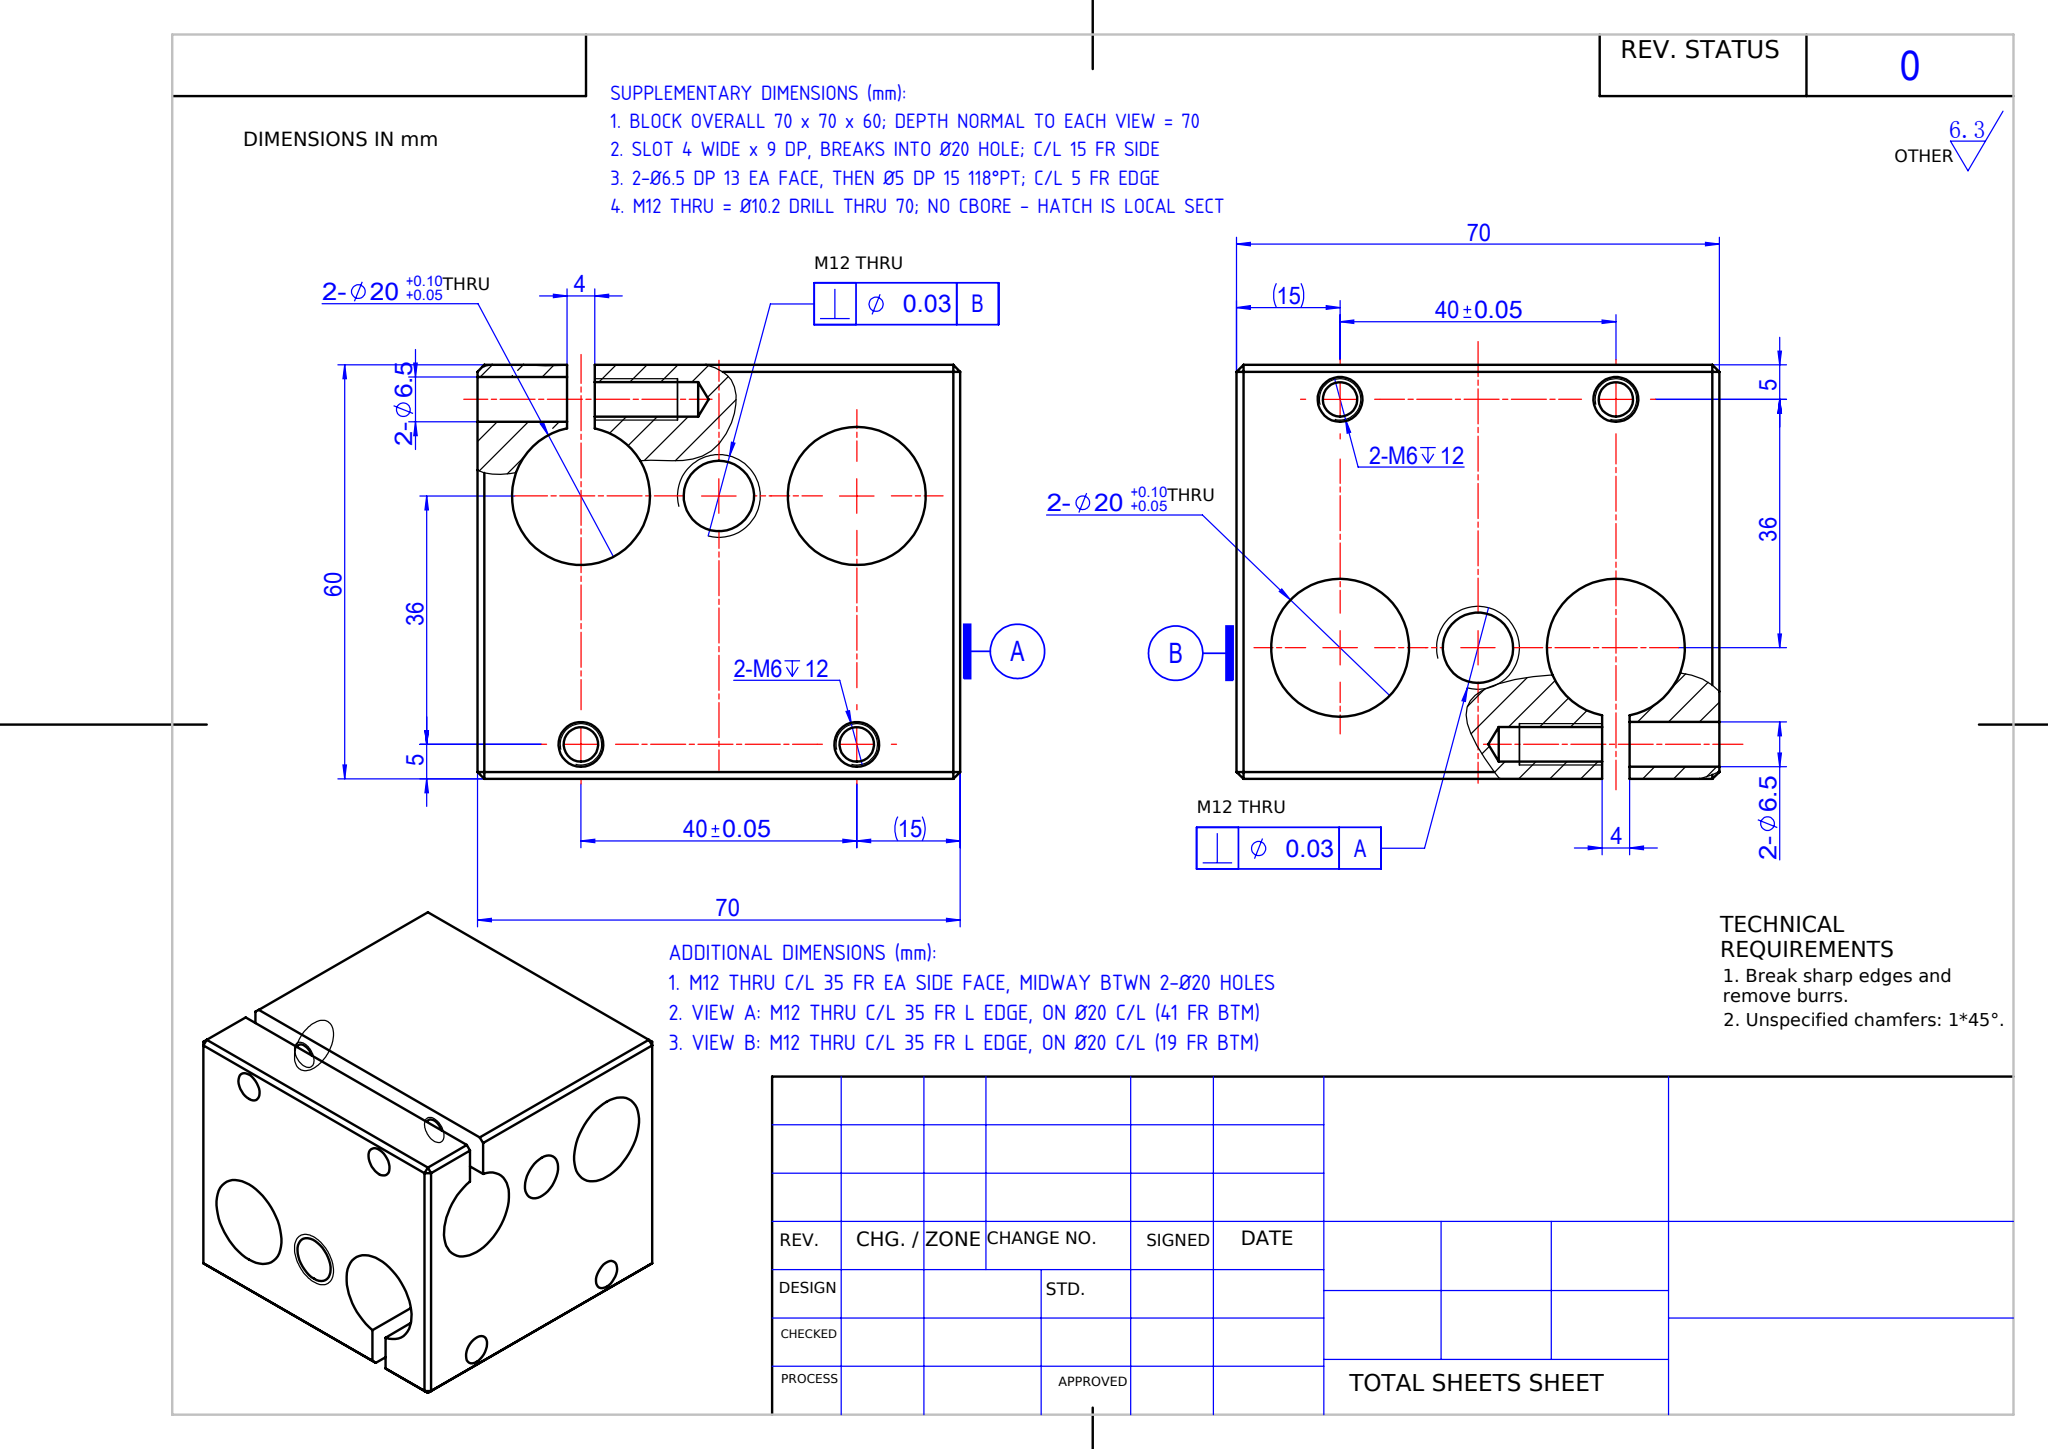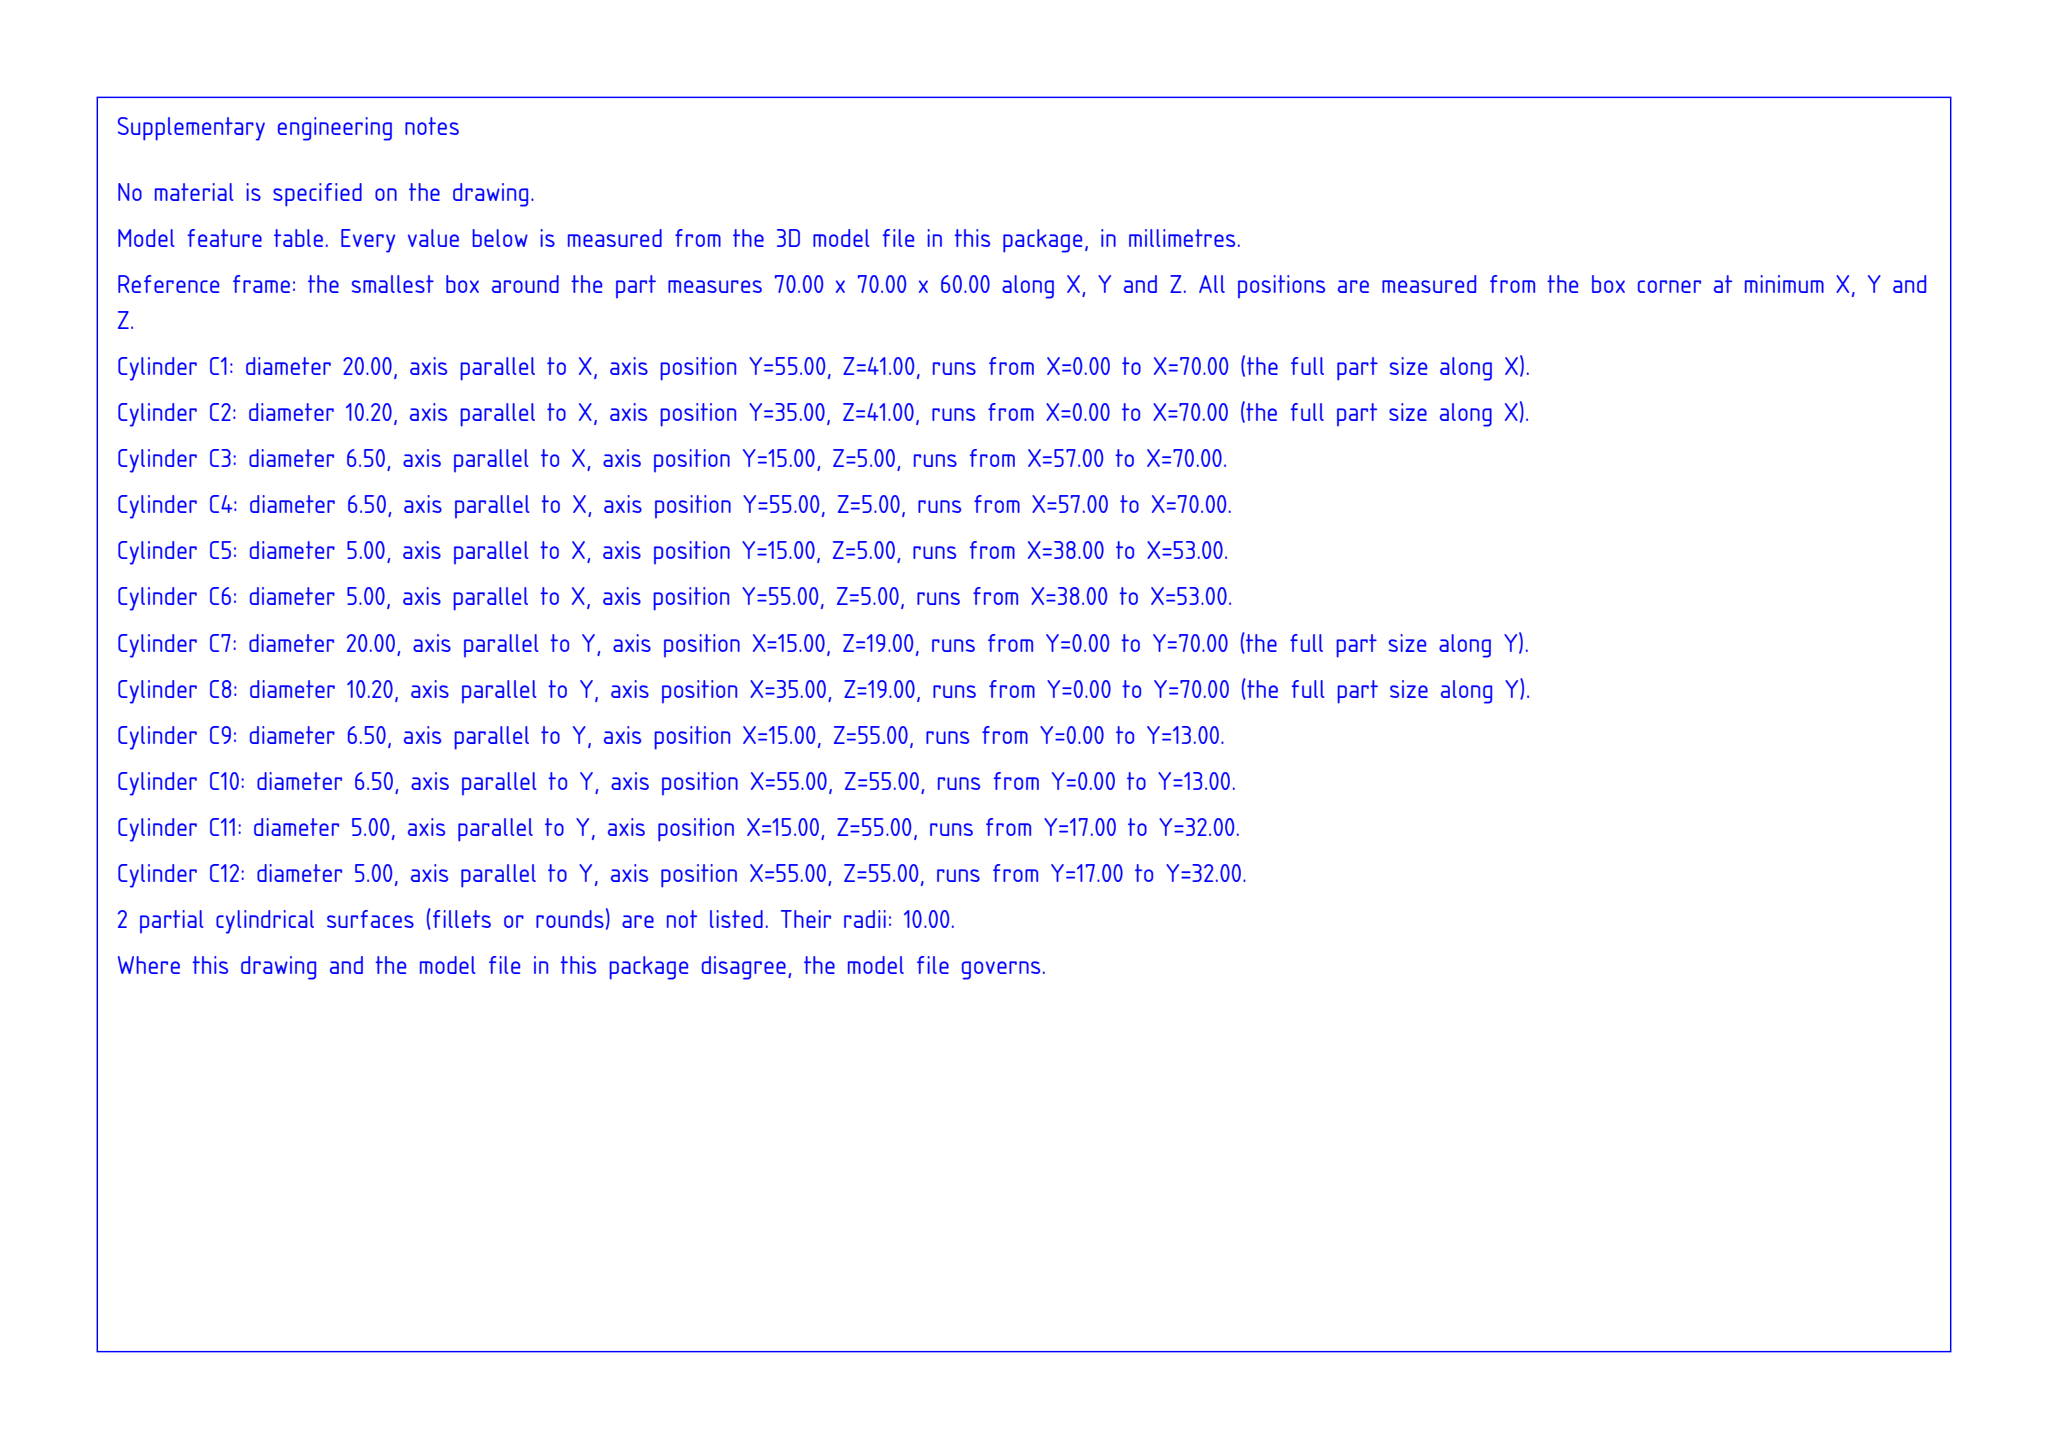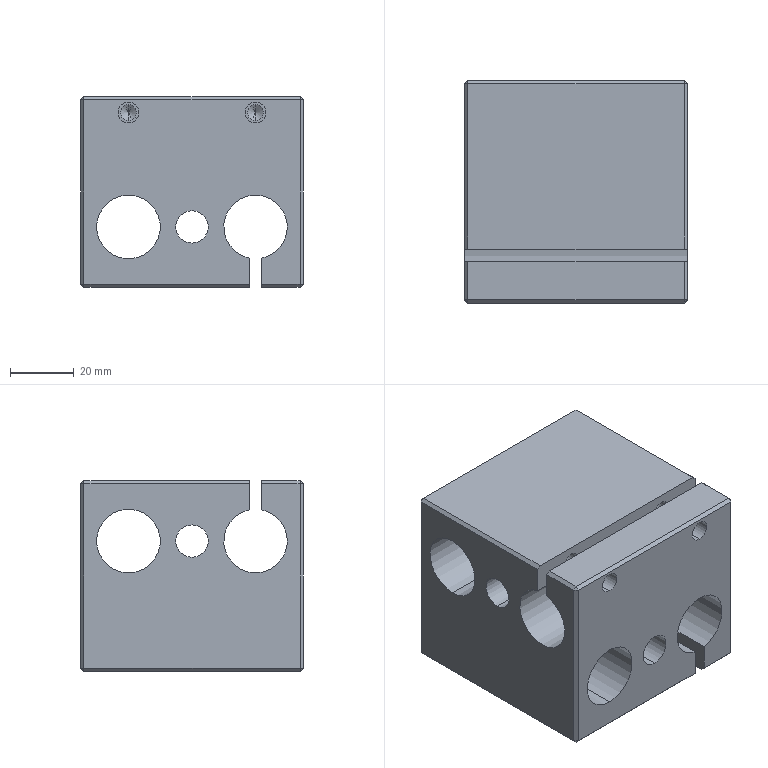Part | SolidWorks | mm | 1 solid | 70 faces | box 70 x 70 x 60 mm | volume 186188 mm3 | plane 36 | cylinder 26 | cone 8 | commonest cylinder face diameters 5 x8 6.5 x8 20 x6 10.2 x4